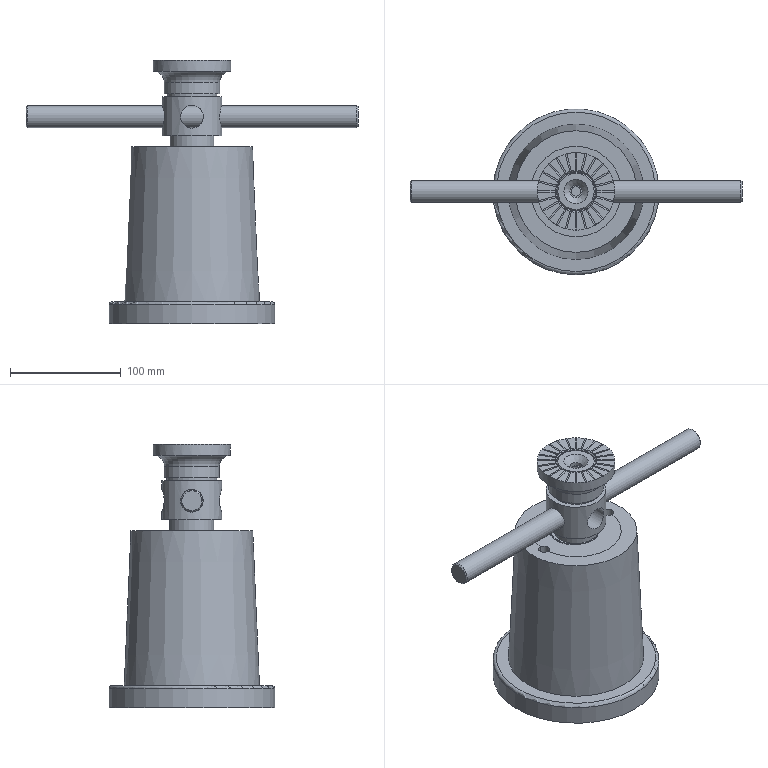Assembly | NX | mm | 6 component files | 6 solids | 119 faces | box 300 x 150 x 238 mm | volume 1435543 mm3 | cylinder 56 | plane 46 | cone 11 | spline 4 | torus 2 | commonest cylinder face diameters 2 x24 82 x4 10 x4 20.5 x4 50 x3 25 x2 65 x2 42 x2
Bill of materials:
unnamed part 1 | 1 |  | Long cylindrical stud. Most of its length has a helical external thread, and one end has a larger cylindrical collar with cross holes. Above the collar is a short, smaller-diameter pin with a small axial hole.
unnamed part 2 | 1 |  | Hollow, tapered cylindrical sleeve with a thin flange around the larger base end and a through bore.
unnamed part 3 | 1 |  | Flanged, bushing-like ring: a wide disc flange with radial ribs on its face, joined by a concave fillet to a smaller cylindrical hub, with a stepped through bore.
unnamed part 4 | 1 |  | Flat, thick annular washer with a conical countersink on one face leading to a smaller cylindrical through hole.
unnamed part 5 | 1 |  | Plain solid cylindrical rod or pin, long relative to its diameter, with flat ends and small edge chamfers or rounds.
unnamed part 6 | 1 |  | Flanged, threaded insert or bushing: a cylindrical body with a larger-diameter flange at one end, an internally threaded through bore, and two diametrically opposed semicircular notches in the flange rim.
Mates:
1. fix | base 1 component
2. concentric | screw_sleeve 1 edge | base 1 edge
3. concentric | lead_screw 1 edge | base 1 edge
4. concentric | top_pad 1 edge | lead_screw 1 edge
5. concentric | end_cap 1 edge | top_pad 1 edge